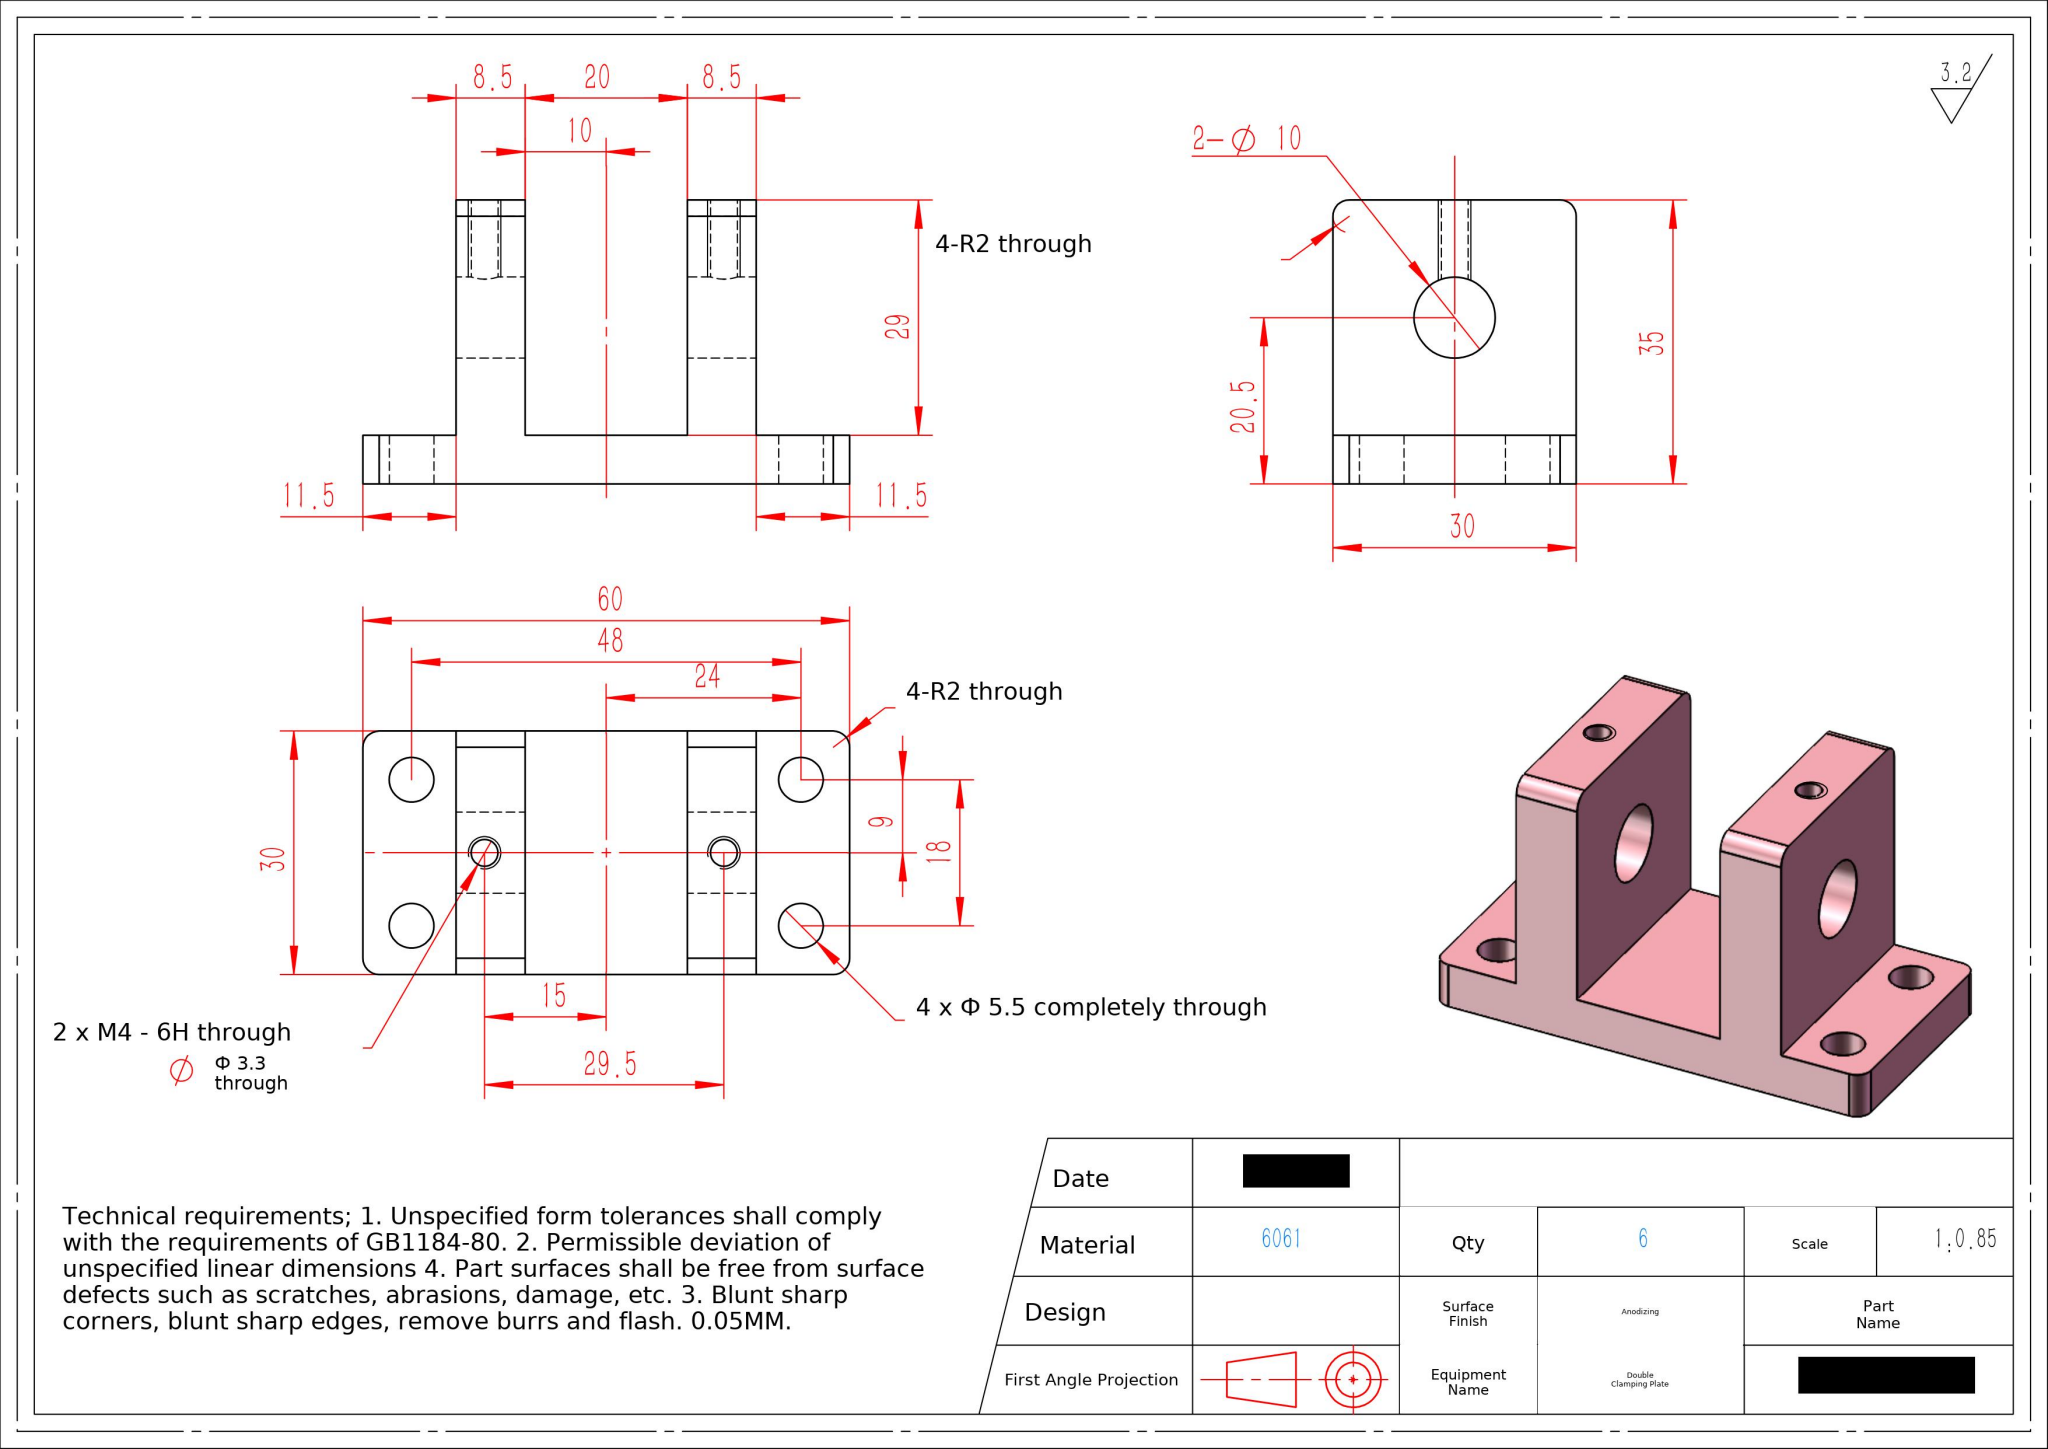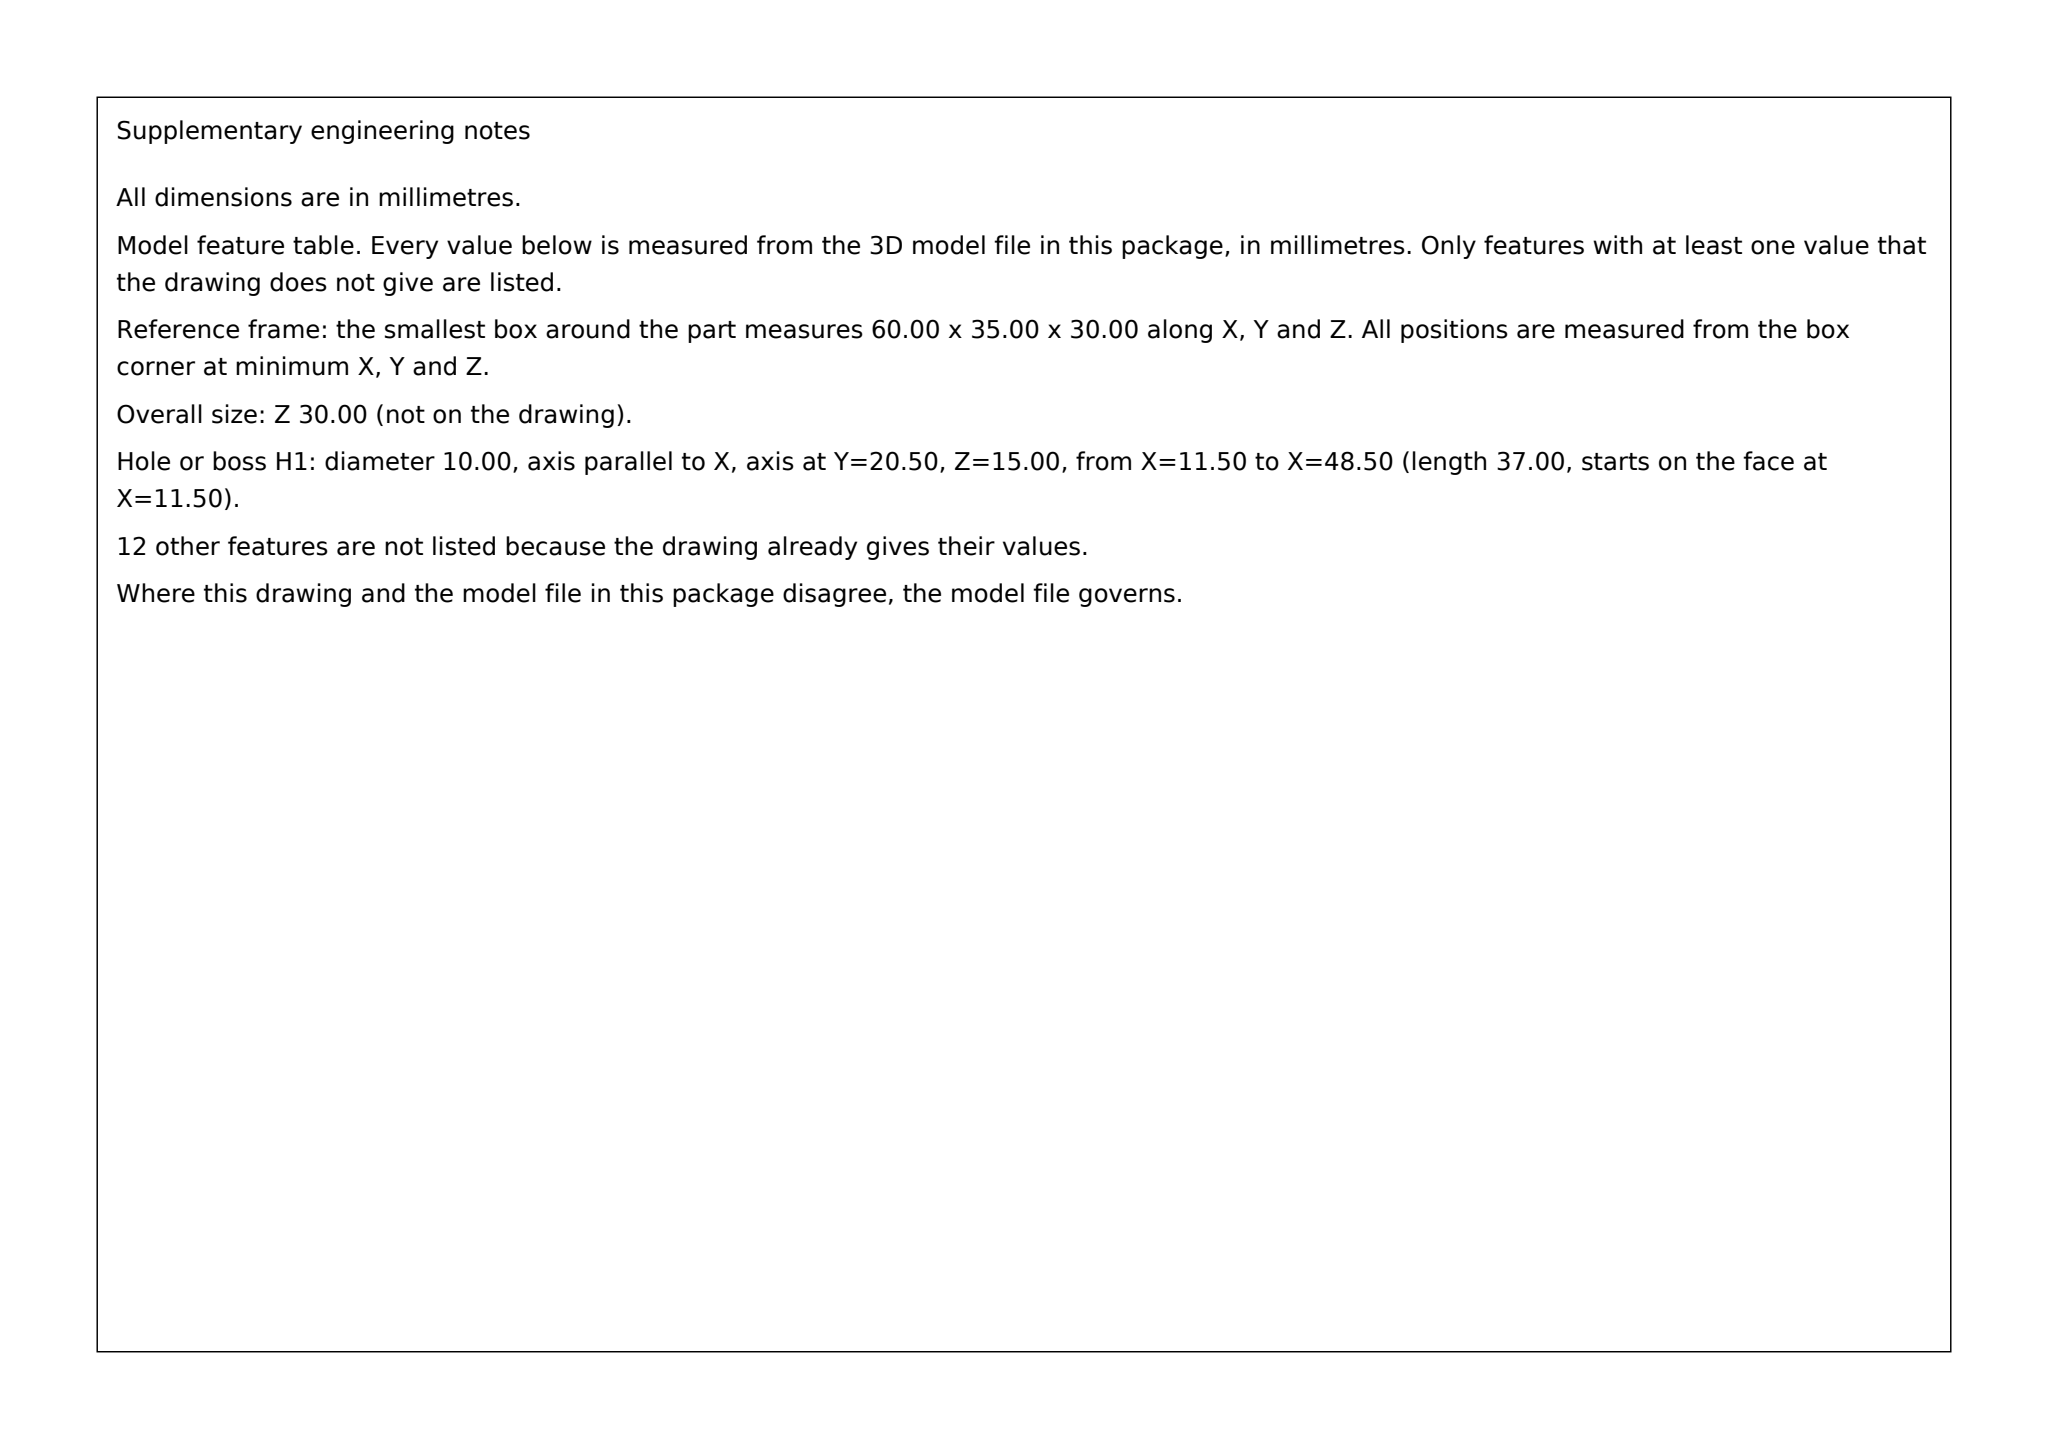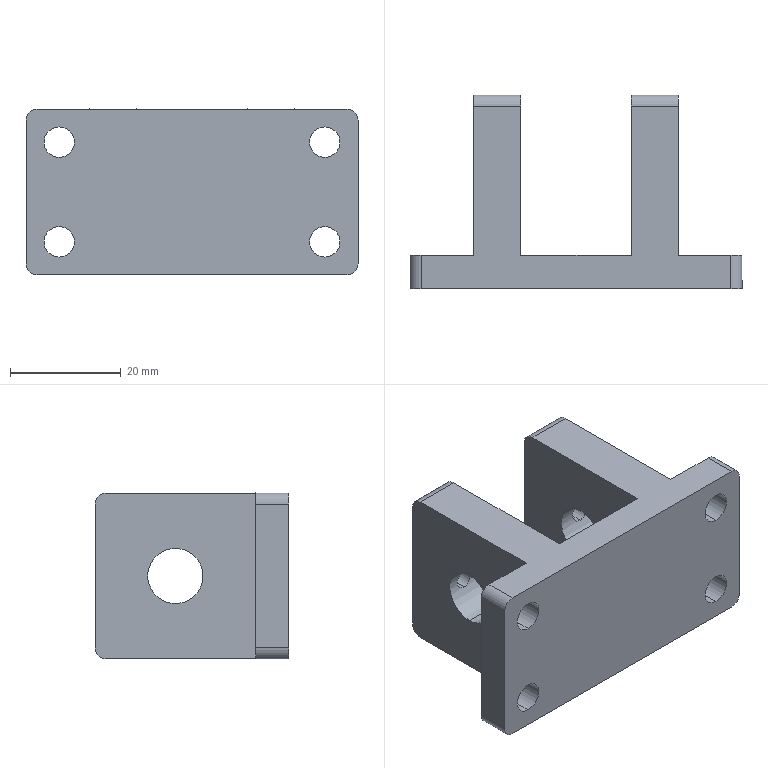Part | SolidWorks | mm | material 6061 | 1 solid | 38 faces | box 60 x 35 x 30 mm | volume 23471 mm3 | cylinder 24 | plane 14 | commonest cylinder face diameters 5.5 x8 4 x8 3.3 x4 10 x4
build123d program:
from build123d import *

# Parameters (mm, degrees)
SKETCH1_W                      = 60
SKETCH1_H                      = 35
BOSS_EXTRUDE1_DEPTH            = 15
SKETCH2_W                      = 11.5
SKETCH2_H                      = 29
CUT_EXTRUDE1_DEPTH             = 46.894
SKETCH3_W                      = 20
SKETCH3_H                      = 29
CUT_EXTRUDE2_DEPTH             = 46.894
SKETCH4_W                      = 11.5
SKETCH4_H                      = 29
CUT_EXTRUDE3_DEPTH             = 46.894
F_10_0_10_DIAMETER_HOLE1_D     = 10
F_10_0_10_DIAMETER_HOLE1_DEPTH = 45.5
M4_TAPPED_HOLE1_REACH          = 57
M4_TAPPED_HOLE1_BORE_R         = 1.65
F_5_5_5_5_DIAMETER_HOLE1_D     = 5.5
FILLET1_R                      = 2


with BuildPart() as part:
    # Sketch1 → Boss-Extrude1 (new, symmetric)
    with BuildSketch(Plane.XY.offset(15)):
        Rectangle(SKETCH1_W, SKETCH1_H)
    extrude(amount=BOSS_EXTRUDE1_DEPTH, both=True)

    # Sketch2 → Cut-Extrude1 (cut, through all)
    with BuildSketch(Plane(origin=(0, 0, 0), x_dir=(-1, 0, 0), z_dir=(0, 0, -1))):
        with Locations((-24.25, 3)):
            Rectangle(SKETCH2_W, SKETCH2_H)
    extrude(amount=-CUT_EXTRUDE1_DEPTH, mode=Mode.SUBTRACT)

    # Sketch3 → Cut-Extrude2 (cut, through all)
    with BuildSketch(Plane(origin=(0, 0, 0), x_dir=(-1, 0, 0), z_dir=(0, 0, -1))):
        with Locations((0, 3)):
            Rectangle(SKETCH3_W, SKETCH3_H)
    extrude(amount=-CUT_EXTRUDE2_DEPTH, mode=Mode.SUBTRACT)

    # Sketch4 → Cut-Extrude3 (cut, through all)
    with BuildSketch(Plane(origin=(0, 0, 0), x_dir=(-1, 0, 0), z_dir=(0, 0, -1))):
        with Locations((24.25, 3)):
            Rectangle(SKETCH4_W, SKETCH4_H)
    extrude(amount=-CUT_EXTRUDE3_DEPTH, mode=Mode.SUBTRACT)

    # 10.0 _10_ Diameter Hole1
    with Locations(Plane(origin=(18.5, 0, 0), x_dir=(0, 0, -1), z_dir=(1, 0, 0))):
        with Locations((-15, 3)):
            Hole(F_10_0_10_DIAMETER_HOLE1_D / 2, depth=F_10_0_10_DIAMETER_HOLE1_DEPTH)

    # M4 Tapped Hole1 bore → M4 Tapped Hole1 (cut, up to next)
    with BuildSketch(Plane(origin=(0, 17.5, 0), x_dir=(1, 0, 0), z_dir=(0, 1, 0)), mode=Mode.PRIVATE) as m4_tapped_hole1_sk1:
        with Locations((14.5, -15)):
            Circle(M4_TAPPED_HOLE1_BORE_R)
    m4_tapped_hole1_tool1 = extrude(m4_tapped_hole1_sk1.sketch, amount=-M4_TAPPED_HOLE1_REACH, mode=Mode.PRIVATE) & part.part
    # M4 Tapped Hole1 bore → M4 Tapped Hole1 (cut, up to next)
    with BuildSketch(Plane(origin=(0, 17.5, 0), x_dir=(1, 0, 0), z_dir=(0, 1, 0)), mode=Mode.PRIVATE) as m4_tapped_hole1_sk2:
        with Locations((-15, -15)):
            Circle(M4_TAPPED_HOLE1_BORE_R)
    m4_tapped_hole1_tool2 = extrude(m4_tapped_hole1_sk2.sketch, amount=-M4_TAPPED_HOLE1_REACH, mode=Mode.PRIVATE) & part.part
    add(m4_tapped_hole1_tool1.solids().sort_by_distance((14.5, 17.5, 15))[0], mode=Mode.SUBTRACT)
    add(m4_tapped_hole1_tool2.solids().sort_by_distance((-15, 17.5, 15))[0], mode=Mode.SUBTRACT)

    # 5.5 _5.5_ Diameter Hole1 (through all)
    with Locations(Plane(origin=(0, -17.5, 0), x_dir=(-1, 0, 0), z_dir=(0, -1, 0))):
        with Locations((-24, -6), (-24, -24), (24, -24), (24, -6)):
            Hole(F_5_5_5_5_DIAMETER_HOLE1_D / 2)

    # Fillet1
    fillet1_edges = [part.edges().sort_by_distance(p)[0] for p in [
        (14.25, 17.5, 30),
        (14.25, 17.5, 0),
        (-14.25, 17.5, 30),
        (-14.25, 17.5, 0),
        (-30, -14.5, 30),
        (-30, -14.5, 0),
        (30, -14.5, 30),
        (30, -14.5, 0),
    ]]
    fillet(fillet1_edges, radius=FILLET1_R)


solid = part.part